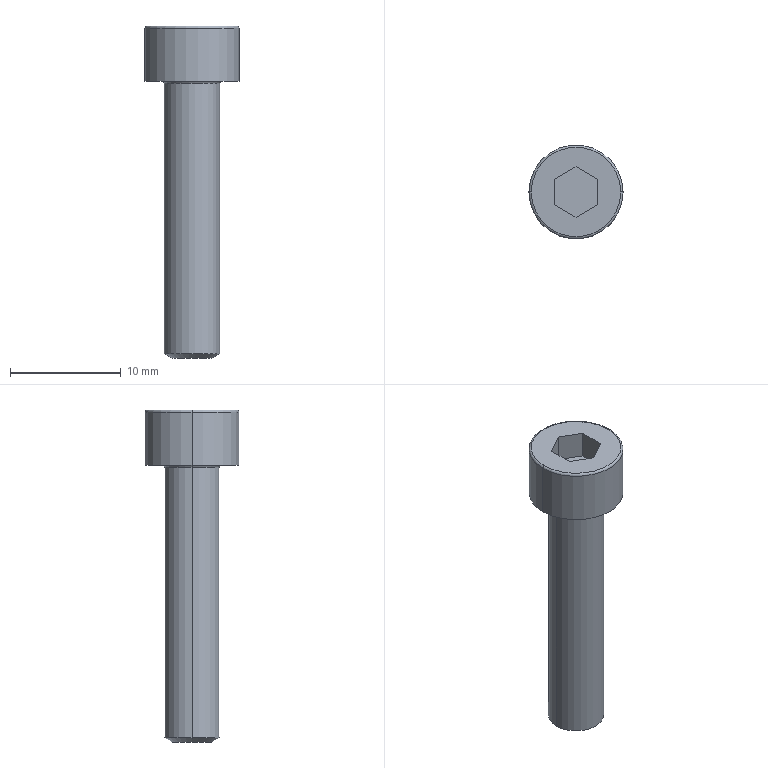Component | NX | HEX_SOCKET_CAP_SCREW_M5X25_2 | 1 solid | 20 faces | volume 738 mm3 | plane 10 | torus 4 | cylinder 4 | cone 2 | commonest cylinder face diameters 8.5 x2 5 x2